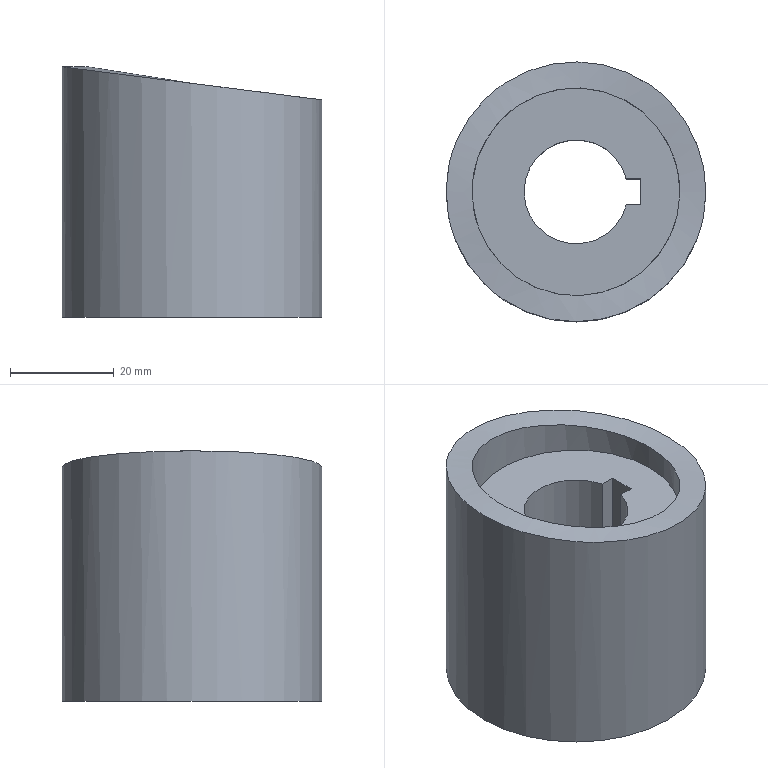Component | NX | CAM | 1 solid | 11 faces | box 50 x 50 x 48.15 mm | volume 54142 mm3 | plane 6 | cylinder 4 | spline 1 | commonest cylinder face diameters 40 x2 50 x1 20 x1
STEP:
#1=CARTESIAN_POINT('',(0.,0.,0.));
#2=DIRECTION('',(0.,0.,1.));
#3=DIRECTION('',(1.,0.,0.));
#4=AXIS2_PLACEMENT_3D('',#1,#2,#3);
#5=CARTESIAN_POINT('',(9.682,-2.5,187.));
#6=VERTEX_POINT('',#5);
#7=CARTESIAN_POINT('',(9.682,2.5,187.));
#8=VERTEX_POINT('',#7);
#9=CARTESIAN_POINT('',(0.,0.,187.));
#10=DIRECTION('',(0.,0.,-1.));
#11=DIRECTION('',(1.,0.,0.));
#12=AXIS2_PLACEMENT_3D('',#9,#10,#11);
#13=CIRCLE('',#12,10.);
#14=CARTESIAN_POINT('',(0.,0.,187.));
#15=DIRECTION('',(0.,0.,1.));
#16=DIRECTION('',(1.,0.,0.));
#17=AXIS2_PLACEMENT_3D('',#14,#15,#16);
#18=PLANE('',#17);
#19=CARTESIAN_POINT('',(10.,0.));
#20=CARTESIAN_POINT('',(10.,-17.321));
#21=CARTESIAN_POINT('',(-5.,-8.66));
#22=CARTESIAN_POINT('',(-20.,-0.));
#23=CARTESIAN_POINT('',(-5.,8.66));
#24=CARTESIAN_POINT('',(10.,17.321));
#25=CARTESIAN_POINT('',(10.,0.));
#26=(BOUNDED_CURVE()B_SPLINE_CURVE(2,(#19,#20,#21,#22,#23,#24,#25),.UNSPECIFIED.,.T.,.F.)B_SPLINE_CURVE_WITH_KNOTS((1,2,2,2,2,1),(-2.094,0.,2.094,4.189,6.283,8.378),.UNSPECIFIED.)CURVE()GEOMETRIC_REPRESENTATION_ITEM()RATIONAL_B_SPLINE_CURVE((1.,0.5,1.,0.5,1.,0.5,1.))REPRESENTATION_ITEM(''));
#27=(GEOMETRIC_REPRESENTATION_CONTEXT(2)PARAMETRIC_REPRESENTATION_CONTEXT()REPRESENTATION_CONTEXT('',''));
#28=DEFINITIONAL_REPRESENTATION('',(#26),#27);
#29=PCURVE('',#18,#28);
#30=CARTESIAN_POINT('',(0.,0.,187.));
#31=DIRECTION('',(0.,0.,-1.));
#32=DIRECTION('',(-1.,0.,0.));
#33=AXIS2_PLACEMENT_3D('',#30,#31,#32);
#34=CYLINDRICAL_SURFACE('',#33,10.);
#35=CARTESIAN_POINT('',(3.142,0.));
#36=DIRECTION('',(1.,0.));
#37=VECTOR('',#36,1.);
#38=LINE('',#35,#37);
#39=(GEOMETRIC_REPRESENTATION_CONTEXT(2)PARAMETRIC_REPRESENTATION_CONTEXT()REPRESENTATION_CONTEXT('',''));
#40=DEFINITIONAL_REPRESENTATION('',(#38),#39);
#41=PCURVE('',#34,#40);
#42=SURFACE_CURVE('',#13,(#29,#41),.PCURVE_S1.);
#43=EDGE_CURVE('',#6,#8,#42,.T.);
#44=ORIENTED_EDGE('',*,*,#43,.T.);
#45=CARTESIAN_POINT('',(12.5,2.5,187.));
#46=VERTEX_POINT('',#45);
#47=CARTESIAN_POINT('',(9.682,2.5,187.));
#48=DIRECTION('',(1.,0.,0.));
#49=VECTOR('',#48,1.);
#50=LINE('',#47,#49);
#51=CARTESIAN_POINT('',(9.682,2.5));
#52=DIRECTION('',(1.,0.));
#53=VECTOR('',#52,1.);
#54=LINE('',#51,#53);
#55=(GEOMETRIC_REPRESENTATION_CONTEXT(2)PARAMETRIC_REPRESENTATION_CONTEXT()REPRESENTATION_CONTEXT('',''));
#56=DEFINITIONAL_REPRESENTATION('',(#54),#55);
#57=PCURVE('',#18,#56);
#58=CARTESIAN_POINT('',(9.682,2.5,187.));
#59=DIRECTION('',(-0.,1.,0.));
#60=DIRECTION('',(-1.,-0.,0.));
#61=AXIS2_PLACEMENT_3D('',#58,#59,#60);
#62=PLANE('',#61);
#63=CARTESIAN_POINT('',(0.,0.));
#64=DIRECTION('',(-1.,0.));
#65=VECTOR('',#64,1.);
#66=LINE('',#63,#65);
#67=(GEOMETRIC_REPRESENTATION_CONTEXT(2)PARAMETRIC_REPRESENTATION_CONTEXT()REPRESENTATION_CONTEXT('',''));
#68=DEFINITIONAL_REPRESENTATION('',(#66),#67);
#69=PCURVE('',#62,#68);
#70=SURFACE_CURVE('',#50,(#57,#69),.PCURVE_S1.);
#71=EDGE_CURVE('',#8,#46,#70,.T.);
#72=ORIENTED_EDGE('',*,*,#71,.T.);
#73=CARTESIAN_POINT('',(12.5,-2.5,187.));
#74=VERTEX_POINT('',#73);
#75=CARTESIAN_POINT('',(12.5,2.5,187.));
#76=DIRECTION('',(0.,-1.,0.));
#77=VECTOR('',#76,1.);
#78=LINE('',#75,#77);
#79=CARTESIAN_POINT('',(12.5,2.5));
#80=DIRECTION('',(0.,-1.));
#81=VECTOR('',#80,1.);
#82=LINE('',#79,#81);
#83=(GEOMETRIC_REPRESENTATION_CONTEXT(2)PARAMETRIC_REPRESENTATION_CONTEXT()REPRESENTATION_CONTEXT('',''));
#84=DEFINITIONAL_REPRESENTATION('',(#82),#83);
#85=PCURVE('',#18,#84);
#86=CARTESIAN_POINT('',(12.5,2.5,187.));
#87=DIRECTION('',(1.,0.,0.));
#88=DIRECTION('',(0.,0.,-1.));
#89=AXIS2_PLACEMENT_3D('',#86,#87,#88);
#90=PLANE('',#89);
#91=CARTESIAN_POINT('',(0.,0.));
#92=DIRECTION('',(0.,-1.));
#93=VECTOR('',#92,1.);
#94=LINE('',#91,#93);
#95=(GEOMETRIC_REPRESENTATION_CONTEXT(2)PARAMETRIC_REPRESENTATION_CONTEXT()REPRESENTATION_CONTEXT('',''));
#96=DEFINITIONAL_REPRESENTATION('',(#94),#95);
#97=PCURVE('',#90,#96);
#98=SURFACE_CURVE('',#78,(#85,#97),.PCURVE_S1.);
#99=EDGE_CURVE('',#46,#74,#98,.T.);
#100=ORIENTED_EDGE('',*,*,#99,.T.);
#101=CARTESIAN_POINT('',(12.5,-2.5,187.));
#102=DIRECTION('',(-1.,0.,0.));
#103=VECTOR('',#102,1.);
#104=LINE('',#101,#103);
#105=CARTESIAN_POINT('',(12.5,-2.5));
#106=DIRECTION('',(-1.,0.));
#107=VECTOR('',#106,1.);
#108=LINE('',#105,#107);
#109=(GEOMETRIC_REPRESENTATION_CONTEXT(2)PARAMETRIC_REPRESENTATION_CONTEXT()REPRESENTATION_CONTEXT('',''));
#110=DEFINITIONAL_REPRESENTATION('',(#108),#109);
#111=PCURVE('',#18,#110);
#112=CARTESIAN_POINT('',(12.5,-2.5,187.));
#113=DIRECTION('',(-0.,-1.,0.));
#114=DIRECTION('',(1.,-0.,0.));
#115=AXIS2_PLACEMENT_3D('',#112,#113,#114);
#116=PLANE('',#115);
#117=CARTESIAN_POINT('',(0.,0.));
#118=DIRECTION('',(-1.,0.));
#119=VECTOR('',#118,1.);
#120=LINE('',#117,#119);
#121=(GEOMETRIC_REPRESENTATION_CONTEXT(2)PARAMETRIC_REPRESENTATION_CONTEXT()REPRESENTATION_CONTEXT('',''));
#122=DEFINITIONAL_REPRESENTATION('',(#120),#121);
#123=PCURVE('',#116,#122);
#124=SURFACE_CURVE('',#104,(#111,#123),.PCURVE_S1.);
#125=EDGE_CURVE('',#74,#6,#124,.T.);
#126=ORIENTED_EDGE('',*,*,#125,.T.);
#127=EDGE_LOOP('',(#44,#72,#100,#126));
#128=FACE_BOUND('',#127,.T.);
#129=CARTESIAN_POINT('',(20.,0.,187.));
#130=VERTEX_POINT('',#129);
#131=CARTESIAN_POINT('',(0.,0.,187.));
#132=DIRECTION('',(0.,0.,1.));
#133=DIRECTION('',(1.,0.,0.));
#134=AXIS2_PLACEMENT_3D('',#131,#132,#133);
#135=CIRCLE('',#134,20.);
#136=CARTESIAN_POINT('',(0.,0.));
#137=DIRECTION('',(1.,0.));
#138=AXIS2_PLACEMENT_2D('',#136,#137);
#139=CIRCLE('',#138,20.);
#140=(GEOMETRIC_REPRESENTATION_CONTEXT(2)PARAMETRIC_REPRESENTATION_CONTEXT()REPRESENTATION_CONTEXT('',''));
#141=DEFINITIONAL_REPRESENTATION('',(#139),#140);
#142=PCURVE('',#18,#141);
#143=CARTESIAN_POINT('',(0.,0.,200.));
#144=DIRECTION('',(0.,0.,-1.));
#145=DIRECTION('',(-1.,0.,0.));
#146=AXIS2_PLACEMENT_3D('',#143,#144,#145);
#147=CYLINDRICAL_SURFACE('',#146,20.);
#148=CARTESIAN_POINT('',(9.425,13.));
#149=DIRECTION('',(-1.,0.));
#150=VECTOR('',#149,1.);
#151=LINE('',#148,#150);
#152=(GEOMETRIC_REPRESENTATION_CONTEXT(2)PARAMETRIC_REPRESENTATION_CONTEXT()REPRESENTATION_CONTEXT('',''));
#153=DEFINITIONAL_REPRESENTATION('',(#151),#152);
#154=PCURVE('',#147,#153);
#155=SURFACE_CURVE('',#135,(#142,#154),.PCURVE_S1.);
#156=EDGE_CURVE('',#130,#130,#155,.T.);
#157=ORIENTED_EDGE('',*,*,#156,.T.);
#158=EDGE_LOOP('',(#157));
#159=FACE_BOUND('',#158,.T.);
#160=ADVANCED_FACE('',(#128,#159),#18,.T.);
#161=CARTESIAN_POINT('',(20.,0.,150.));
#162=VERTEX_POINT('',#161);
#163=CARTESIAN_POINT('',(0.,0.,150.));
#164=DIRECTION('',(0.,0.,1.));
#165=DIRECTION('',(1.,0.,0.));
#166=AXIS2_PLACEMENT_3D('',#163,#164,#165);
#167=CIRCLE('',#166,20.);
#168=CARTESIAN_POINT('',(0.,0.,200.));
#169=DIRECTION('',(0.,0.,-1.));
#170=DIRECTION('',(-1.,0.,0.));
#171=AXIS2_PLACEMENT_3D('',#168,#169,#170);
#172=CYLINDRICAL_SURFACE('',#171,20.);
#173=CARTESIAN_POINT('',(9.425,50.));
#174=DIRECTION('',(-1.,0.));
#175=VECTOR('',#174,1.);
#176=LINE('',#173,#175);
#177=(GEOMETRIC_REPRESENTATION_CONTEXT(2)PARAMETRIC_REPRESENTATION_CONTEXT()REPRESENTATION_CONTEXT('',''));
#178=DEFINITIONAL_REPRESENTATION('',(#176),#177);
#179=PCURVE('',#172,#178);
#180=CARTESIAN_POINT('',(0.,0.,150.));
#181=DIRECTION('',(0.,0.,1.));
#182=DIRECTION('',(1.,0.,0.));
#183=AXIS2_PLACEMENT_3D('',#180,#181,#182);
#184=PLANE('',#183);
#185=CARTESIAN_POINT('',(0.,0.));
#186=DIRECTION('',(1.,0.));
#187=AXIS2_PLACEMENT_2D('',#185,#186);
#188=CIRCLE('',#187,20.);
#189=(GEOMETRIC_REPRESENTATION_CONTEXT(2)PARAMETRIC_REPRESENTATION_CONTEXT()REPRESENTATION_CONTEXT('',''));
#190=DEFINITIONAL_REPRESENTATION('',(#188),#189);
#191=PCURVE('',#184,#190);
#192=SURFACE_CURVE('',#167,(#179,#191),.PCURVE_S1.);
#193=EDGE_CURVE('',#162,#162,#192,.T.);
#194=ORIENTED_EDGE('',*,*,#193,.T.);
#195=CARTESIAN_POINT('',(20.,0.,163.));
#196=VERTEX_POINT('',#195);
#197=CARTESIAN_POINT('',(20.,0.,163.));
#198=CARTESIAN_POINT('',(20.,0.,150.));
#199=B_SPLINE_CURVE_WITH_KNOTS('',1,(#197,#198),.UNSPECIFIED.,.F.,.F.,(2,2),(37.,50.),.PIECEWISE_BEZIER_KNOTS.);
#200=CARTESIAN_POINT('',(3.142,0.));
#201=DIRECTION('',(0.,1.));
#202=VECTOR('',#201,1.);
#203=LINE('',#200,#202);
#204=(GEOMETRIC_REPRESENTATION_CONTEXT(2)PARAMETRIC_REPRESENTATION_CONTEXT()REPRESENTATION_CONTEXT('',''));
#205=DEFINITIONAL_REPRESENTATION('',(#203),#204);
#206=PCURVE('',#172,#205);
#207=CARTESIAN_POINT('',(9.425,0.));
#208=DIRECTION('',(0.,1.));
#209=VECTOR('',#208,1.);
#210=LINE('',#207,#209);
#211=(GEOMETRIC_REPRESENTATION_CONTEXT(2)PARAMETRIC_REPRESENTATION_CONTEXT()REPRESENTATION_CONTEXT('',''));
#212=DEFINITIONAL_REPRESENTATION('',(#210),#211);
#213=PCURVE('',#172,#212);
#214=SEAM_CURVE('',#199,(#206,#213),.PCURVE_S1.);
#215=EDGE_CURVE('',#196,#162,#214,.T.);
#216=ORIENTED_EDGE('',*,*,#215,.F.);
#217=CARTESIAN_POINT('',(0.,0.,163.));
#218=DIRECTION('',(0.,0.,1.));
#219=DIRECTION('',(1.,0.,0.));
#220=AXIS2_PLACEMENT_3D('',#217,#218,#219);
#221=CIRCLE('',#220,20.);
#222=CARTESIAN_POINT('',(9.425,37.));
#223=DIRECTION('',(-1.,0.));
#224=VECTOR('',#223,1.);
#225=LINE('',#222,#224);
#226=(GEOMETRIC_REPRESENTATION_CONTEXT(2)PARAMETRIC_REPRESENTATION_CONTEXT()REPRESENTATION_CONTEXT('',''));
#227=DEFINITIONAL_REPRESENTATION('',(#225),#226);
#228=PCURVE('',#172,#227);
#229=CARTESIAN_POINT('',(0.,0.,163.));
#230=DIRECTION('',(0.,0.,1.));
#231=DIRECTION('',(1.,0.,0.));
#232=AXIS2_PLACEMENT_3D('',#229,#230,#231);
#233=PLANE('',#232);
#234=CARTESIAN_POINT('',(0.,0.));
#235=DIRECTION('',(1.,0.));
#236=AXIS2_PLACEMENT_2D('',#234,#235);
#237=CIRCLE('',#236,20.);
#238=(GEOMETRIC_REPRESENTATION_CONTEXT(2)PARAMETRIC_REPRESENTATION_CONTEXT()REPRESENTATION_CONTEXT('',''));
#239=DEFINITIONAL_REPRESENTATION('',(#237),#238);
#240=PCURVE('',#233,#239);
#241=SURFACE_CURVE('',#221,(#228,#240),.PCURVE_S1.);
#242=EDGE_CURVE('',#196,#196,#241,.T.);
#243=ORIENTED_EDGE('',*,*,#242,.F.);
#244=ORIENTED_EDGE('',*,*,#215,.T.);
#245=EDGE_LOOP('',(#194,#216,#243,#244));
#246=FACE_BOUND('',#245,.F.);
#247=ADVANCED_FACE('',(#246),#172,.F.);
#248=CARTESIAN_POINT('',(25.,0.,150.));
#249=VERTEX_POINT('',#248);
#250=CARTESIAN_POINT('',(0.,0.,150.));
#251=DIRECTION('',(0.,0.,1.));
#252=DIRECTION('',(1.,0.,0.));
#253=AXIS2_PLACEMENT_3D('',#250,#251,#252);
#254=CIRCLE('',#253,25.);
#255=CARTESIAN_POINT('',(0.,0.,200.));
#256=DIRECTION('',(0.,0.,-1.));
#257=DIRECTION('',(-1.,0.,0.));
#258=AXIS2_PLACEMENT_3D('',#255,#256,#257);
#259=CYLINDRICAL_SURFACE('',#258,25.);
#260=CARTESIAN_POINT('',(9.425,50.));
#261=DIRECTION('',(-1.,0.));
#262=VECTOR('',#261,1.);
#263=LINE('',#260,#262);
#264=(GEOMETRIC_REPRESENTATION_CONTEXT(2)PARAMETRIC_REPRESENTATION_CONTEXT()REPRESENTATION_CONTEXT('',''));
#265=DEFINITIONAL_REPRESENTATION('',(#263),#264);
#266=PCURVE('',#259,#265);
#267=CARTESIAN_POINT('',(0.,0.));
#268=DIRECTION('',(1.,0.));
#269=AXIS2_PLACEMENT_2D('',#267,#268);
#270=CIRCLE('',#269,25.);
#271=(GEOMETRIC_REPRESENTATION_CONTEXT(2)PARAMETRIC_REPRESENTATION_CONTEXT()REPRESENTATION_CONTEXT('',''));
#272=DEFINITIONAL_REPRESENTATION('',(#270),#271);
#273=PCURVE('',#184,#272);
#274=SURFACE_CURVE('',#254,(#266,#273),.PCURVE_S1.);
#275=EDGE_CURVE('',#249,#249,#274,.T.);
#276=ORIENTED_EDGE('',*,*,#275,.T.);
#277=CARTESIAN_POINT('',(25.,0.,191.818));
#278=VERTEX_POINT('',#277);
#279=CARTESIAN_POINT('',(25.,0.,191.818));
#280=CARTESIAN_POINT('',(25.,0.,150.));
#281=B_SPLINE_CURVE_WITH_KNOTS('',1,(#279,#280),.UNSPECIFIED.,.F.,.F.,(2,2),(8.182,50.),.PIECEWISE_BEZIER_KNOTS.);
#282=CARTESIAN_POINT('',(3.142,0.));
#283=DIRECTION('',(0.,1.));
#284=VECTOR('',#283,1.);
#285=LINE('',#282,#284);
#286=(GEOMETRIC_REPRESENTATION_CONTEXT(2)PARAMETRIC_REPRESENTATION_CONTEXT()REPRESENTATION_CONTEXT('',''));
#287=DEFINITIONAL_REPRESENTATION('',(#285),#286);
#288=PCURVE('',#259,#287);
#289=CARTESIAN_POINT('',(9.425,0.));
#290=DIRECTION('',(0.,1.));
#291=VECTOR('',#290,1.);
#292=LINE('',#289,#291);
#293=(GEOMETRIC_REPRESENTATION_CONTEXT(2)PARAMETRIC_REPRESENTATION_CONTEXT()REPRESENTATION_CONTEXT('',''));
#294=DEFINITIONAL_REPRESENTATION('',(#292),#293);
#295=PCURVE('',#259,#294);
#296=SEAM_CURVE('',#281,(#288,#295),.PCURVE_S1.);
#297=EDGE_CURVE('',#278,#249,#296,.T.);
#298=ORIENTED_EDGE('',*,*,#297,.F.);
#299=CARTESIAN_POINT('',(0.,0.,194.986));
#300=DIRECTION('',(-0.1257,0.,-0.9921));
#301=DIRECTION('',(0.9921,0.,-0.1257));
#302=AXIS2_PLACEMENT_3D('',#299,#300,#301);
#303=ELLIPSE('',#302,25.2,25.);
#304=CARTESIAN_POINT('',(3.142,8.182));
#305=CARTESIAN_POINT('',(3.237,8.183));
#306=CARTESIAN_POINT('',(3.427,8.094));
#307=CARTESIAN_POINT('',(3.713,7.715));
#308=CARTESIAN_POINT('',(3.998,7.117));
#309=CARTESIAN_POINT('',(4.284,6.348));
#310=CARTESIAN_POINT('',(4.57,5.471));
#311=CARTESIAN_POINT('',(4.855,4.557));
#312=CARTESIAN_POINT('',(5.141,3.68));
#313=CARTESIAN_POINT('',(5.426,2.911));
#314=CARTESIAN_POINT('',(5.712,2.313));
#315=CARTESIAN_POINT('',(5.998,1.933));
#316=CARTESIAN_POINT('',(6.283,1.803));
#317=CARTESIAN_POINT('',(6.569,1.933));
#318=CARTESIAN_POINT('',(6.854,2.313));
#319=CARTESIAN_POINT('',(7.14,2.911));
#320=CARTESIAN_POINT('',(7.426,3.68));
#321=CARTESIAN_POINT('',(7.711,4.557));
#322=CARTESIAN_POINT('',(7.997,5.471));
#323=CARTESIAN_POINT('',(8.282,6.348));
#324=CARTESIAN_POINT('',(8.568,7.117));
#325=CARTESIAN_POINT('',(8.854,7.715));
#326=CARTESIAN_POINT('',(9.139,8.094));
#327=CARTESIAN_POINT('',(9.33,8.183));
#328=CARTESIAN_POINT('',(9.425,8.182));
#329=B_SPLINE_CURVE_WITH_KNOTS('',3,(#304,#305,#306,#307,#308,#309,#310,#311,#312,#313,#314,#315,#316,#317,#318,#319,#320,#321,#322,#323,#324,#325,#326,#327,#328),.UNSPECIFIED.,.F.,.F.,(4,1,1,1,1,1,1,1,1,1,1,1,1,1,1,1,1,1,1,1,1,1,4),(0.,0.2856,0.5712,0.8568,1.142,1.428,1.714,1.999,2.285,2.57,2.856,3.142,3.427,3.713,3.998,4.284,4.57,4.855,5.141,5.426,5.712,5.998,6.283),.QUASI_UNIFORM_KNOTS.);
#330=(GEOMETRIC_REPRESENTATION_CONTEXT(2)PARAMETRIC_REPRESENTATION_CONTEXT()REPRESENTATION_CONTEXT('',''));
#331=DEFINITIONAL_REPRESENTATION('',(#329),#330);
#332=PCURVE('',#259,#331);
#333=CARTESIAN_POINT('',(20.,0.,191.818));
#334=CARTESIAN_POINT('',(21.667,0.,191.818));
#335=CARTESIAN_POINT('',(23.333,0.,191.818));
#336=CARTESIAN_POINT('',(25.,0.,191.818));
#337=CARTESIAN_POINT('',(20.,-40.,191.818));
#338=CARTESIAN_POINT('',(21.667,-43.333,191.818));
#339=CARTESIAN_POINT('',(23.333,-46.667,191.818));
#340=CARTESIAN_POINT('',(25.,-50.,191.818));
#341=CARTESIAN_POINT('',(-20.,-40.,198.154));
#342=CARTESIAN_POINT('',(-21.667,-43.333,198.154));
#343=CARTESIAN_POINT('',(-23.333,-46.667,198.154));
#344=CARTESIAN_POINT('',(-25.,-50.,198.154));
#345=CARTESIAN_POINT('',(-20.,-0.,198.154));
#346=CARTESIAN_POINT('',(-21.667,-0.,198.154));
#347=CARTESIAN_POINT('',(-23.333,-0.,198.154));
#348=CARTESIAN_POINT('',(-25.,-0.,198.154));
#349=CARTESIAN_POINT('',(-20.,40.,198.154));
#350=CARTESIAN_POINT('',(-21.667,43.333,198.154));
#351=CARTESIAN_POINT('',(-23.333,46.667,198.154));
#352=CARTESIAN_POINT('',(-25.,50.,198.154));
#353=CARTESIAN_POINT('',(20.,40.,191.818));
#354=CARTESIAN_POINT('',(21.667,43.333,191.818));
#355=CARTESIAN_POINT('',(23.333,46.667,191.818));
#356=CARTESIAN_POINT('',(25.,50.,191.818));
#357=CARTESIAN_POINT('',(20.,0.,191.818));
#358=CARTESIAN_POINT('',(21.667,0.,191.818));
#359=CARTESIAN_POINT('',(23.333,0.,191.818));
#360=CARTESIAN_POINT('',(25.,0.,191.818));
#361=(BOUNDED_SURFACE()B_SPLINE_SURFACE(3,3,((#333,#334,#335,#336),(#337,#338,#339,#340),(#341,#342,#343,#344),(#345,#346,#347,#348),(#349,#350,#351,#352),(#353,#354,#355,#356),(#357,#358,#359,#360)),.UNSPECIFIED.,.T.,.F.,.F.)B_SPLINE_SURFACE_WITH_KNOTS((1,3,3,3,1),(4,4),(-0.5,0.,0.5,1.,1.5),(0.,1.),.UNSPECIFIED.)GEOMETRIC_REPRESENTATION_ITEM()RATIONAL_B_SPLINE_SURFACE(((1.,1.,1.,1.),(0.3333,0.3333,0.3333,0.3333),(0.3333,0.3333,0.3333,0.3333),(1.,1.,1.,1.),(0.3333,0.3333,0.3333,0.3333),(0.3333,0.3333,0.3333,0.3333),(1.,1.,1.,1.)))REPRESENTATION_ITEM('')SURFACE());
#362=CARTESIAN_POINT('',(0.,1.));
#363=CARTESIAN_POINT('',(0.02352,1.));
#364=CARTESIAN_POINT('',(0.06491,1.));
#365=CARTESIAN_POINT('',(0.1146,1.));
#366=CARTESIAN_POINT('',(0.1575,1.));
#367=CARTESIAN_POINT('',(0.196,1.));
#368=CARTESIAN_POINT('',(0.2322,1.));
#369=CARTESIAN_POINT('',(0.2678,1.));
#370=CARTESIAN_POINT('',(0.304,1.));
#371=CARTESIAN_POINT('',(0.3425,1.));
#372=CARTESIAN_POINT('',(0.3856,1.));
#373=CARTESIAN_POINT('',(0.4343,1.));
#374=CARTESIAN_POINT('',(0.5,1.));
#375=CARTESIAN_POINT('',(0.5657,1.));
#376=CARTESIAN_POINT('',(0.6144,1.));
#377=CARTESIAN_POINT('',(0.6575,1.));
#378=CARTESIAN_POINT('',(0.696,1.));
#379=CARTESIAN_POINT('',(0.7322,1.));
#380=CARTESIAN_POINT('',(0.7678,1.));
#381=CARTESIAN_POINT('',(0.804,1.));
#382=CARTESIAN_POINT('',(0.8425,1.));
#383=CARTESIAN_POINT('',(0.8854,1.));
#384=CARTESIAN_POINT('',(0.9351,1.));
#385=CARTESIAN_POINT('',(0.9765,1.));
#386=CARTESIAN_POINT('',(1.,1.));
#387=B_SPLINE_CURVE_WITH_KNOTS('',3,(#362,#363,#364,#365,#366,#367,#368,#369,#370,#371,#372,#373,#374,#375,#376,#377,#378,#379,#380,#381,#382,#383,#384,#385,#386),.UNSPECIFIED.,.F.,.F.,(4,1,1,1,1,1,1,1,1,1,1,1,1,1,1,1,1,1,1,1,1,1,4),(0.,0.2856,0.5712,0.8568,1.142,1.428,1.714,1.999,2.285,2.57,2.856,3.142,3.427,3.713,3.998,4.284,4.57,4.855,5.141,5.426,5.712,5.998,6.283),.QUASI_UNIFORM_KNOTS.);
#388=(GEOMETRIC_REPRESENTATION_CONTEXT(2)PARAMETRIC_REPRESENTATION_CONTEXT()REPRESENTATION_CONTEXT('',''));
#389=DEFINITIONAL_REPRESENTATION('',(#387),#388);
#390=PCURVE('',#361,#389);
#391=SURFACE_CURVE('',#303,(#332,#390),.PCURVE_S1.);
#392=EDGE_CURVE('',#278,#278,#391,.T.);
#393=ORIENTED_EDGE('',*,*,#392,.T.);
#394=ORIENTED_EDGE('',*,*,#297,.T.);
#395=EDGE_LOOP('',(#276,#298,#393,#394));
#396=FACE_BOUND('',#395,.T.);
#397=ADVANCED_FACE('',(#396),#259,.T.);
#398=ORIENTED_EDGE('',*,*,#275,.F.);
#399=EDGE_LOOP('',(#398));
#400=FACE_BOUND('',#399,.T.);
#401=ORIENTED_EDGE('',*,*,#193,.T.);
#402=EDGE_LOOP('',(#401));
#403=FACE_BOUND('',#402,.T.);
#404=ADVANCED_FACE('',(#400,#403),#184,.F.);
#405=CARTESIAN_POINT('',(9.682,-2.5,163.));
#406=VERTEX_POINT('',#405);
#407=CARTESIAN_POINT('',(9.682,-2.5,187.));
#408=DIRECTION('',(0.,0.,-1.));
#409=VECTOR('',#408,1.);
#410=LINE('',#407,#409);
#411=CARTESIAN_POINT('',(3.394,0.));
#412=DIRECTION('',(0.,1.));
#413=VECTOR('',#412,1.);
#414=LINE('',#411,#413);
#415=(GEOMETRIC_REPRESENTATION_CONTEXT(2)PARAMETRIC_REPRESENTATION_CONTEXT()REPRESENTATION_CONTEXT('',''));
#416=DEFINITIONAL_REPRESENTATION('',(#414),#415);
#417=PCURVE('',#34,#416);
#418=CARTESIAN_POINT('',(-2.818,0.));
#419=DIRECTION('',(0.,-1.));
#420=VECTOR('',#419,1.);
#421=LINE('',#418,#420);
#422=(GEOMETRIC_REPRESENTATION_CONTEXT(2)PARAMETRIC_REPRESENTATION_CONTEXT()REPRESENTATION_CONTEXT('',''));
#423=DEFINITIONAL_REPRESENTATION('',(#421),#422);
#424=PCURVE('',#116,#423);
#425=SURFACE_CURVE('',#410,(#417,#424),.PCURVE_S1.);
#426=EDGE_CURVE('',#6,#406,#425,.T.);
#427=ORIENTED_EDGE('',*,*,#426,.F.);
#428=ORIENTED_EDGE('',*,*,#43,.T.);
#429=CARTESIAN_POINT('',(9.682,2.5,163.));
#430=VERTEX_POINT('',#429);
#431=CARTESIAN_POINT('',(9.682,2.5,187.));
#432=DIRECTION('',(0.,0.,-1.));
#433=VECTOR('',#432,1.);
#434=LINE('',#431,#433);
#435=CARTESIAN_POINT('',(9.172,0.));
#436=DIRECTION('',(0.,1.));
#437=VECTOR('',#436,1.);
#438=LINE('',#435,#437);
#439=(GEOMETRIC_REPRESENTATION_CONTEXT(2)PARAMETRIC_REPRESENTATION_CONTEXT()REPRESENTATION_CONTEXT('',''));
#440=DEFINITIONAL_REPRESENTATION('',(#438),#439);
#441=PCURVE('',#34,#440);
#442=CARTESIAN_POINT('',(0.,0.));
#443=DIRECTION('',(0.,-1.));
#444=VECTOR('',#443,1.);
#445=LINE('',#442,#444);
#446=(GEOMETRIC_REPRESENTATION_CONTEXT(2)PARAMETRIC_REPRESENTATION_CONTEXT()REPRESENTATION_CONTEXT('',''));
#447=DEFINITIONAL_REPRESENTATION('',(#445),#446);
#448=PCURVE('',#62,#447);
#449=SURFACE_CURVE('',#434,(#441,#448),.PCURVE_S1.);
#450=EDGE_CURVE('',#8,#430,#449,.T.);
#451=ORIENTED_EDGE('',*,*,#450,.T.);
#452=CARTESIAN_POINT('',(0.,0.,163.));
#453=DIRECTION('',(0.,0.,-1.));
#454=DIRECTION('',(1.,0.,0.));
#455=AXIS2_PLACEMENT_3D('',#452,#453,#454);
#456=CIRCLE('',#455,10.);
#457=CARTESIAN_POINT('',(3.142,24.));
#458=DIRECTION('',(1.,0.));
#459=VECTOR('',#458,1.);
#460=LINE('',#457,#459);
#461=(GEOMETRIC_REPRESENTATION_CONTEXT(2)PARAMETRIC_REPRESENTATION_CONTEXT()REPRESENTATION_CONTEXT('',''));
#462=DEFINITIONAL_REPRESENTATION('',(#460),#461);
#463=PCURVE('',#34,#462);
#464=CARTESIAN_POINT('',(10.,0.));
#465=CARTESIAN_POINT('',(10.,-17.321));
#466=CARTESIAN_POINT('',(-5.,-8.66));
#467=CARTESIAN_POINT('',(-20.,-0.));
#468=CARTESIAN_POINT('',(-5.,8.66));
#469=CARTESIAN_POINT('',(10.,17.321));
#470=CARTESIAN_POINT('',(10.,0.));
#471=(BOUNDED_CURVE()B_SPLINE_CURVE(2,(#464,#465,#466,#467,#468,#469,#470),.UNSPECIFIED.,.T.,.F.)B_SPLINE_CURVE_WITH_KNOTS((1,2,2,2,2,1),(-2.094,0.,2.094,4.189,6.283,8.378),.UNSPECIFIED.)CURVE()GEOMETRIC_REPRESENTATION_ITEM()RATIONAL_B_SPLINE_CURVE((1.,0.5,1.,0.5,1.,0.5,1.))REPRESENTATION_ITEM(''));
#472=(GEOMETRIC_REPRESENTATION_CONTEXT(2)PARAMETRIC_REPRESENTATION_CONTEXT()REPRESENTATION_CONTEXT('',''));
#473=DEFINITIONAL_REPRESENTATION('',(#471),#472);
#474=PCURVE('',#233,#473);
#475=SURFACE_CURVE('',#456,(#463,#474),.PCURVE_S1.);
#476=EDGE_CURVE('',#406,#430,#475,.T.);
#477=ORIENTED_EDGE('',*,*,#476,.F.);
#478=EDGE_LOOP('',(#427,#428,#451,#477));
#479=FACE_BOUND('',#478,.F.);
#480=ADVANCED_FACE('',(#479),#34,.F.);
#481=CARTESIAN_POINT('',(12.5,2.5,163.));
#482=VERTEX_POINT('',#481);
#483=CARTESIAN_POINT('',(9.682,2.5,163.));
#484=DIRECTION('',(1.,0.,0.));
#485=VECTOR('',#484,1.);
#486=LINE('',#483,#485);
#487=CARTESIAN_POINT('',(0.,-24.));
#488=DIRECTION('',(-1.,0.));
#489=VECTOR('',#488,1.);
#490=LINE('',#487,#489);
#491=(GEOMETRIC_REPRESENTATION_CONTEXT(2)PARAMETRIC_REPRESENTATION_CONTEXT()REPRESENTATION_CONTEXT('',''));
#492=DEFINITIONAL_REPRESENTATION('',(#490),#491);
#493=PCURVE('',#62,#492);
#494=CARTESIAN_POINT('',(9.682,2.5));
#495=DIRECTION('',(1.,0.));
#496=VECTOR('',#495,1.);
#497=LINE('',#494,#496);
#498=(GEOMETRIC_REPRESENTATION_CONTEXT(2)PARAMETRIC_REPRESENTATION_CONTEXT()REPRESENTATION_CONTEXT('',''));
#499=DEFINITIONAL_REPRESENTATION('',(#497),#498);
#500=PCURVE('',#233,#499);
#501=SURFACE_CURVE('',#486,(#493,#500),.PCURVE_S1.);
#502=EDGE_CURVE('',#430,#482,#501,.T.);
#503=ORIENTED_EDGE('',*,*,#502,.T.);
#504=CARTESIAN_POINT('',(12.5,2.5,187.));
#505=DIRECTION('',(0.,0.,-1.));
#506=VECTOR('',#505,1.);
#507=LINE('',#504,#506);
#508=CARTESIAN_POINT('',(-2.818,0.));
#509=DIRECTION('',(0.,-1.));
#510=VECTOR('',#509,1.);
#511=LINE('',#508,#510);
#512=(GEOMETRIC_REPRESENTATION_CONTEXT(2)PARAMETRIC_REPRESENTATION_CONTEXT()REPRESENTATION_CONTEXT('',''));
#513=DEFINITIONAL_REPRESENTATION('',(#511),#512);
#514=PCURVE('',#62,#513);
#515=CARTESIAN_POINT('',(0.,0.));
#516=DIRECTION('',(1.,0.));
#517=VECTOR('',#516,1.);
#518=LINE('',#515,#517);
#519=(GEOMETRIC_REPRESENTATION_CONTEXT(2)PARAMETRIC_REPRESENTATION_CONTEXT()REPRESENTATION_CONTEXT('',''));
#520=DEFINITIONAL_REPRESENTATION('',(#518),#519);
#521=PCURVE('',#90,#520);
#522=SURFACE_CURVE('',#507,(#514,#521),.PCURVE_S1.);
#523=EDGE_CURVE('',#46,#482,#522,.T.);
#524=ORIENTED_EDGE('',*,*,#523,.F.);
#525=ORIENTED_EDGE('',*,*,#71,.F.);
#526=ORIENTED_EDGE('',*,*,#450,.T.);
#527=EDGE_LOOP('',(#503,#524,#525,#526));
#528=FACE_BOUND('',#527,.T.);
#529=ADVANCED_FACE('',(#528),#62,.F.);
#530=CARTESIAN_POINT('',(12.5,-2.5,163.));
#531=VERTEX_POINT('',#530);
#532=CARTESIAN_POINT('',(12.5,2.5,163.));
#533=DIRECTION('',(0.,-1.,0.));
#534=VECTOR('',#533,1.);
#535=LINE('',#532,#534);
#536=CARTESIAN_POINT('',(24.,0.));
#537=DIRECTION('',(0.,-1.));
#538=VECTOR('',#537,1.);
#539=LINE('',#536,#538);
#540=(GEOMETRIC_REPRESENTATION_CONTEXT(2)PARAMETRIC_REPRESENTATION_CONTEXT()REPRESENTATION_CONTEXT('',''));
#541=DEFINITIONAL_REPRESENTATION('',(#539),#540);
#542=PCURVE('',#90,#541);
#543=CARTESIAN_POINT('',(12.5,2.5));
#544=DIRECTION('',(0.,-1.));
#545=VECTOR('',#544,1.);
#546=LINE('',#543,#545);
#547=(GEOMETRIC_REPRESENTATION_CONTEXT(2)PARAMETRIC_REPRESENTATION_CONTEXT()REPRESENTATION_CONTEXT('',''));
#548=DEFINITIONAL_REPRESENTATION('',(#546),#547);
#549=PCURVE('',#233,#548);
#550=SURFACE_CURVE('',#535,(#542,#549),.PCURVE_S1.);
#551=EDGE_CURVE('',#482,#531,#550,.T.);
#552=ORIENTED_EDGE('',*,*,#551,.T.);
#553=CARTESIAN_POINT('',(12.5,-2.5,187.));
#554=DIRECTION('',(0.,0.,-1.));
#555=VECTOR('',#554,1.);
#556=LINE('',#553,#555);
#557=CARTESIAN_POINT('',(0.,-5.));
#558=DIRECTION('',(1.,0.));
#559=VECTOR('',#558,1.);
#560=LINE('',#557,#559);
#561=(GEOMETRIC_REPRESENTATION_CONTEXT(2)PARAMETRIC_REPRESENTATION_CONTEXT()REPRESENTATION_CONTEXT('',''));
#562=DEFINITIONAL_REPRESENTATION('',(#560),#561);
#563=PCURVE('',#90,#562);
#564=CARTESIAN_POINT('',(0.,0.));
#565=DIRECTION('',(0.,-1.));
#566=VECTOR('',#565,1.);
#567=LINE('',#564,#566);
#568=(GEOMETRIC_REPRESENTATION_CONTEXT(2)PARAMETRIC_REPRESENTATION_CONTEXT()REPRESENTATION_CONTEXT('',''));
#569=DEFINITIONAL_REPRESENTATION('',(#567),#568);
#570=PCURVE('',#116,#569);
#571=SURFACE_CURVE('',#556,(#563,#570),.PCURVE_S1.);
#572=EDGE_CURVE('',#74,#531,#571,.T.);
#573=ORIENTED_EDGE('',*,*,#572,.F.);
#574=ORIENTED_EDGE('',*,*,#99,.F.);
#575=ORIENTED_EDGE('',*,*,#523,.T.);
#576=EDGE_LOOP('',(#552,#573,#574,#575));
#577=FACE_BOUND('',#576,.T.);
#578=ADVANCED_FACE('',(#577),#90,.F.);
#579=CARTESIAN_POINT('',(12.5,-2.5,163.));
#580=DIRECTION('',(-1.,0.,0.));
#581=VECTOR('',#580,1.);
#582=LINE('',#579,#581);
#583=CARTESIAN_POINT('',(0.,-24.));
#584=DIRECTION('',(-1.,0.));
#585=VECTOR('',#584,1.);
#586=LINE('',#583,#585);
#587=(GEOMETRIC_REPRESENTATION_CONTEXT(2)PARAMETRIC_REPRESENTATION_CONTEXT()REPRESENTATION_CONTEXT('',''));
#588=DEFINITIONAL_REPRESENTATION('',(#586),#587);
#589=PCURVE('',#116,#588);
#590=CARTESIAN_POINT('',(12.5,-2.5));
#591=DIRECTION('',(-1.,0.));
#592=VECTOR('',#591,1.);
#593=LINE('',#590,#592);
#594=(GEOMETRIC_REPRESENTATION_CONTEXT(2)PARAMETRIC_REPRESENTATION_CONTEXT()REPRESENTATION_CONTEXT('',''));
#595=DEFINITIONAL_REPRESENTATION('',(#593),#594);
#596=PCURVE('',#233,#595);
#597=SURFACE_CURVE('',#582,(#589,#596),.PCURVE_S1.);
#598=EDGE_CURVE('',#531,#406,#597,.T.);
#599=ORIENTED_EDGE('',*,*,#598,.T.);
#600=ORIENTED_EDGE('',*,*,#426,.F.);
#601=ORIENTED_EDGE('',*,*,#125,.F.);
#602=ORIENTED_EDGE('',*,*,#572,.T.);
#603=EDGE_LOOP('',(#599,#600,#601,#602));
#604=FACE_BOUND('',#603,.T.);
#605=ADVANCED_FACE('',(#604),#116,.F.);
#606=ORIENTED_EDGE('',*,*,#242,.F.);
#607=EDGE_LOOP('',(#606));
#608=FACE_BOUND('',#607,.T.);
#609=ORIENTED_EDGE('',*,*,#476,.F.);
#610=ORIENTED_EDGE('',*,*,#598,.F.);
#611=ORIENTED_EDGE('',*,*,#551,.F.);
#612=ORIENTED_EDGE('',*,*,#502,.F.);
#613=EDGE_LOOP('',(#609,#610,#611,#612));
#614=FACE_BOUND('',#613,.T.);
#615=ADVANCED_FACE('',(#608,#614),#233,.F.);
#616=ORIENTED_EDGE('',*,*,#392,.F.);
#617=CARTESIAN_POINT('',(20.,0.,191.818));
#618=VERTEX_POINT('',#617);
#619=CARTESIAN_POINT('',(20.,0.,191.818));
#620=CARTESIAN_POINT('',(21.667,0.,191.818));
#621=CARTESIAN_POINT('',(23.333,0.,191.818));
#622=CARTESIAN_POINT('',(25.,0.,191.818));
#623=B_SPLINE_CURVE_WITH_KNOTS('',3,(#619,#620,#621,#622),.UNSPECIFIED.,.F.,.F.,(4,4),(0.,1.),.PIECEWISE_BEZIER_KNOTS.);
#624=CARTESIAN_POINT('',(0.,0.));
#625=DIRECTION('',(0.,1.));
#626=VECTOR('',#625,1.);
#627=LINE('',#624,#626);
#628=(GEOMETRIC_REPRESENTATION_CONTEXT(2)PARAMETRIC_REPRESENTATION_CONTEXT()REPRESENTATION_CONTEXT('',''));
#629=DEFINITIONAL_REPRESENTATION('',(#627),#628);
#630=PCURVE('',#361,#629);
#631=CARTESIAN_POINT('',(1.,0.));
#632=DIRECTION('',(0.,1.));
#633=VECTOR('',#632,1.);
#634=LINE('',#631,#633);
#635=(GEOMETRIC_REPRESENTATION_CONTEXT(2)PARAMETRIC_REPRESENTATION_CONTEXT()REPRESENTATION_CONTEXT('',''));
#636=DEFINITIONAL_REPRESENTATION('',(#634),#635);
#637=PCURVE('',#361,#636);
#638=SEAM_CURVE('',#623,(#630,#637),.PCURVE_S1.);
#639=EDGE_CURVE('',#618,#278,#638,.T.);
#640=ORIENTED_EDGE('',*,*,#639,.F.);
#641=CARTESIAN_POINT('',(0.,0.,194.986));
#642=DIRECTION('',(-0.1564,0.,-0.9877));
#643=DIRECTION('',(0.9877,0.,-0.1564));
#644=AXIS2_PLACEMENT_3D('',#641,#642,#643);
#645=ELLIPSE('',#644,20.249,20.);
#646=CARTESIAN_POINT('',(0.,0.));
#647=CARTESIAN_POINT('',(0.02352,0.));
#648=CARTESIAN_POINT('',(0.06491,0.));
#649=CARTESIAN_POINT('',(0.1146,0.));
#650=CARTESIAN_POINT('',(0.1575,0.));
#651=CARTESIAN_POINT('',(0.196,0.));
#652=CARTESIAN_POINT('',(0.2322,0.));
#653=CARTESIAN_POINT('',(0.2678,0.));
#654=CARTESIAN_POINT('',(0.304,0.));
#655=CARTESIAN_POINT('',(0.3425,0.));
#656=CARTESIAN_POINT('',(0.3856,0.));
#657=CARTESIAN_POINT('',(0.4343,0.));
#658=CARTESIAN_POINT('',(0.5,0.));
#659=CARTESIAN_POINT('',(0.5657,0.));
#660=CARTESIAN_POINT('',(0.6144,0.));
#661=CARTESIAN_POINT('',(0.6575,0.));
#662=CARTESIAN_POINT('',(0.696,0.));
#663=CARTESIAN_POINT('',(0.7322,0.));
#664=CARTESIAN_POINT('',(0.7678,0.));
#665=CARTESIAN_POINT('',(0.804,0.));
#666=CARTESIAN_POINT('',(0.8425,0.));
#667=CARTESIAN_POINT('',(0.8854,0.));
#668=CARTESIAN_POINT('',(0.9351,0.));
#669=CARTESIAN_POINT('',(0.9765,0.));
#670=CARTESIAN_POINT('',(1.,0.));
#671=B_SPLINE_CURVE_WITH_KNOTS('',3,(#646,#647,#648,#649,#650,#651,#652,#653,#654,#655,#656,#657,#658,#659,#660,#661,#662,#663,#664,#665,#666,#667,#668,#669,#670),.UNSPECIFIED.,.F.,.F.,(4,1,1,1,1,1,1,1,1,1,1,1,1,1,1,1,1,1,1,1,1,1,4),(0.,0.2856,0.5712,0.8568,1.142,1.428,1.714,1.999,2.285,2.57,2.856,3.142,3.427,3.713,3.998,4.284,4.57,4.855,5.141,5.426,5.712,5.998,6.283),.QUASI_UNIFORM_KNOTS.);
#672=(GEOMETRIC_REPRESENTATION_CONTEXT(2)PARAMETRIC_REPRESENTATION_CONTEXT()REPRESENTATION_CONTEXT('',''));
#673=DEFINITIONAL_REPRESENTATION('',(#671),#672);
#674=PCURVE('',#361,#673);
#675=CARTESIAN_POINT('',(3.142,8.182));
#676=CARTESIAN_POINT('',(3.237,8.183));
#677=CARTESIAN_POINT('',(3.427,8.094));
#678=CARTESIAN_POINT('',(3.713,7.715));
#679=CARTESIAN_POINT('',(3.998,7.117));
#680=CARTESIAN_POINT('',(4.284,6.348));
#681=CARTESIAN_POINT('',(4.57,5.471));
#682=CARTESIAN_POINT('',(4.855,4.557));
#683=CARTESIAN_POINT('',(5.141,3.68));
#684=CARTESIAN_POINT('',(5.426,2.911));
#685=CARTESIAN_POINT('',(5.712,2.313));
#686=CARTESIAN_POINT('',(5.998,1.933));
#687=CARTESIAN_POINT('',(6.283,1.803));
#688=CARTESIAN_POINT('',(6.569,1.933));
#689=CARTESIAN_POINT('',(6.854,2.313));
#690=CARTESIAN_POINT('',(7.14,2.911));
#691=CARTESIAN_POINT('',(7.426,3.68));
#692=CARTESIAN_POINT('',(7.711,4.557));
#693=CARTESIAN_POINT('',(7.997,5.471));
#694=CARTESIAN_POINT('',(8.282,6.348));
#695=CARTESIAN_POINT('',(8.568,7.117));
#696=CARTESIAN_POINT('',(8.854,7.715));
#697=CARTESIAN_POINT('',(9.139,8.094));
#698=CARTESIAN_POINT('',(9.33,8.183));
#699=CARTESIAN_POINT('',(9.425,8.182));
#700=B_SPLINE_CURVE_WITH_KNOTS('',3,(#675,#676,#677,#678,#679,#680,#681,#682,#683,#684,#685,#686,#687,#688,#689,#690,#691,#692,#693,#694,#695,#696,#697,#698,#699),.UNSPECIFIED.,.F.,.F.,(4,1,1,1,1,1,1,1,1,1,1,1,1,1,1,1,1,1,1,1,1,1,4),(0.,0.2856,0.5712,0.8568,1.142,1.428,1.714,1.999,2.285,2.57,2.856,3.142,3.427,3.713,3.998,4.284,4.57,4.855,5.141,5.426,5.712,5.998,6.283),.QUASI_UNIFORM_KNOTS.);
#701=(GEOMETRIC_REPRESENTATION_CONTEXT(2)PARAMETRIC_REPRESENTATION_CONTEXT()REPRESENTATION_CONTEXT('',''));
#702=DEFINITIONAL_REPRESENTATION('',(#700),#701);
#703=PCURVE('',#147,#702);
#704=SURFACE_CURVE('',#645,(#674,#703),.PCURVE_S1.);
#705=EDGE_CURVE('',#618,#618,#704,.T.);
#706=ORIENTED_EDGE('',*,*,#705,.T.);
#707=ORIENTED_EDGE('',*,*,#639,.T.);
#708=EDGE_LOOP('',(#616,#640,#706,#707));
#709=FACE_BOUND('',#708,.T.);
#710=ADVANCED_FACE('',(#709),#361,.T.);
#711=ORIENTED_EDGE('',*,*,#705,.T.);
#712=CARTESIAN_POINT('',(20.,0.,191.818));
#713=CARTESIAN_POINT('',(20.,0.,187.));
#714=B_SPLINE_CURVE_WITH_KNOTS('',1,(#712,#713),.UNSPECIFIED.,.F.,.F.,(2,2),(8.182,13.),.PIECEWISE_BEZIER_KNOTS.);
#715=CARTESIAN_POINT('',(9.425,0.));
#716=DIRECTION('',(0.,1.));
#717=VECTOR('',#716,1.);
#718=LINE('',#715,#717);
#719=(GEOMETRIC_REPRESENTATION_CONTEXT(2)PARAMETRIC_REPRESENTATION_CONTEXT()REPRESENTATION_CONTEXT('',''));
#720=DEFINITIONAL_REPRESENTATION('',(#718),#719);
#721=PCURVE('',#147,#720);
#722=CARTESIAN_POINT('',(3.142,0.));
#723=DIRECTION('',(0.,1.));
#724=VECTOR('',#723,1.);
#725=LINE('',#722,#724);
#726=(GEOMETRIC_REPRESENTATION_CONTEXT(2)PARAMETRIC_REPRESENTATION_CONTEXT()REPRESENTATION_CONTEXT('',''));
#727=DEFINITIONAL_REPRESENTATION('',(#725),#726);
#728=PCURVE('',#147,#727);
#729=SEAM_CURVE('',#714,(#721,#728),.PCURVE_S1.);
#730=EDGE_CURVE('',#618,#130,#729,.T.);
#731=ORIENTED_EDGE('',*,*,#730,.T.);
#732=ORIENTED_EDGE('',*,*,#156,.T.);
#733=ORIENTED_EDGE('',*,*,#730,.F.);
#734=EDGE_LOOP('',(#711,#731,#732,#733));
#735=FACE_BOUND('',#734,.F.);
#736=ADVANCED_FACE('',(#735),#147,.F.);
#737=CLOSED_SHELL('',(#160,#247,#397,#404,#480,#529,#578,#605,#615,#710,#736));
#738=MANIFOLD_SOLID_BREP('',#737);
#739=(LENGTH_UNIT()NAMED_UNIT(*)SI_UNIT(.MILLI.,.METRE.));
#740=UNCERTAINTY_MEASURE_WITH_UNIT(LENGTH_MEASURE(0.000005),#739,'','');
#741=(NAMED_UNIT(*)PLANE_ANGLE_UNIT()SI_UNIT($,.RADIAN.));
#742=(NAMED_UNIT(*)SI_UNIT($,.STERADIAN.)SOLID_ANGLE_UNIT());
#743=(GEOMETRIC_REPRESENTATION_CONTEXT(3)GLOBAL_UNCERTAINTY_ASSIGNED_CONTEXT((#740))GLOBAL_UNIT_ASSIGNED_CONTEXT((#739,#741,#742))REPRESENTATION_CONTEXT('',''));
#744=ADVANCED_BREP_SHAPE_REPRESENTATION('',(#4,#738),#743);